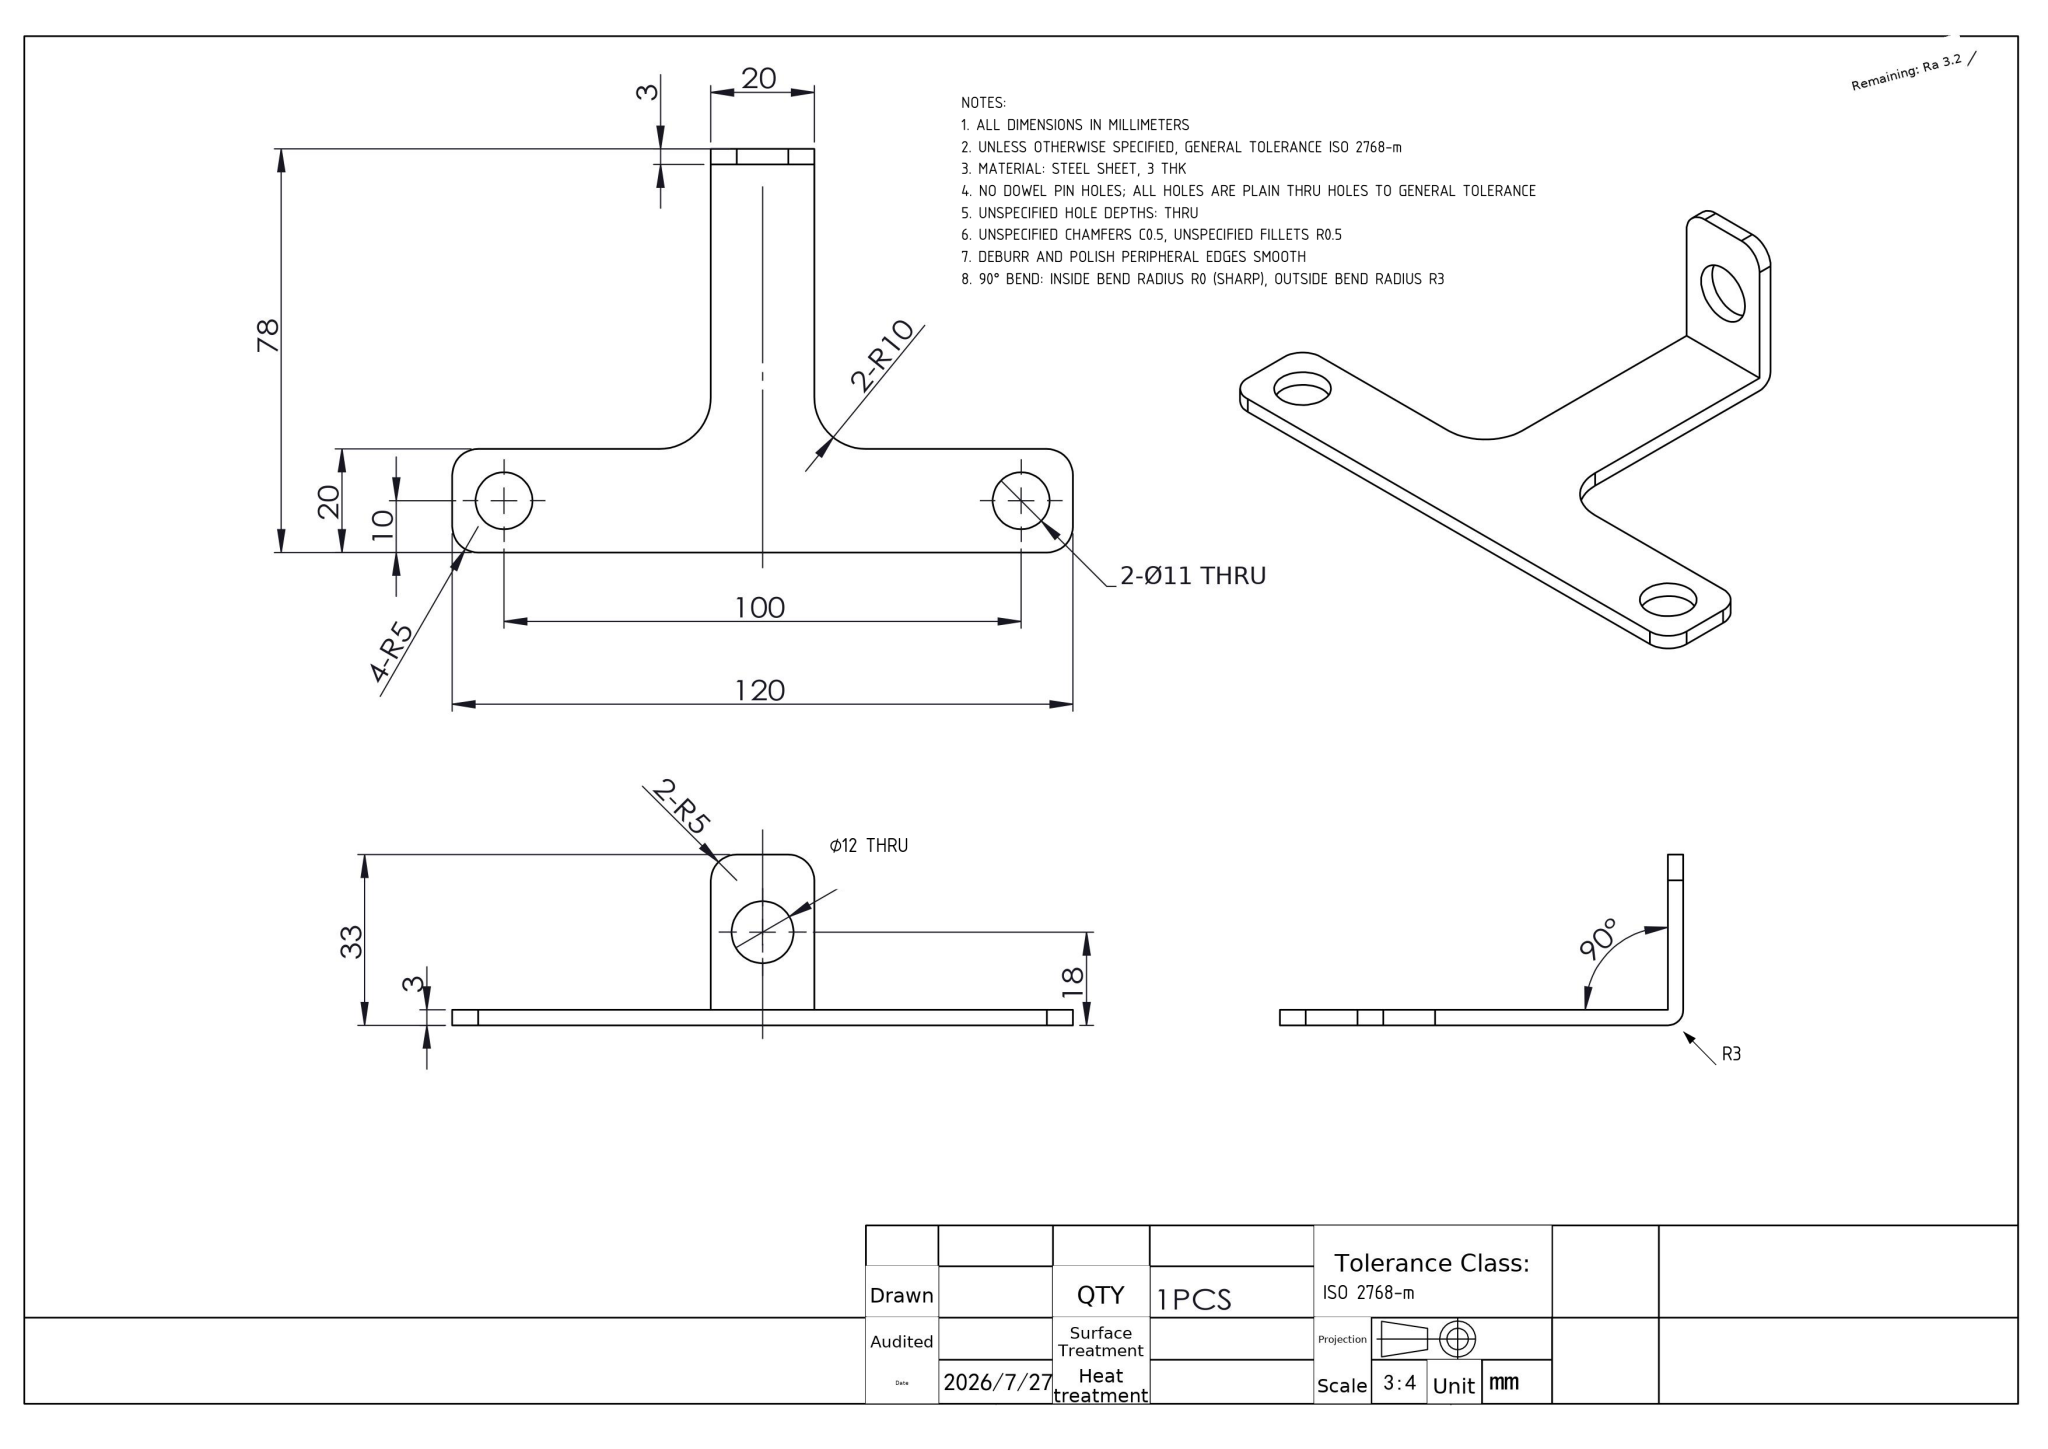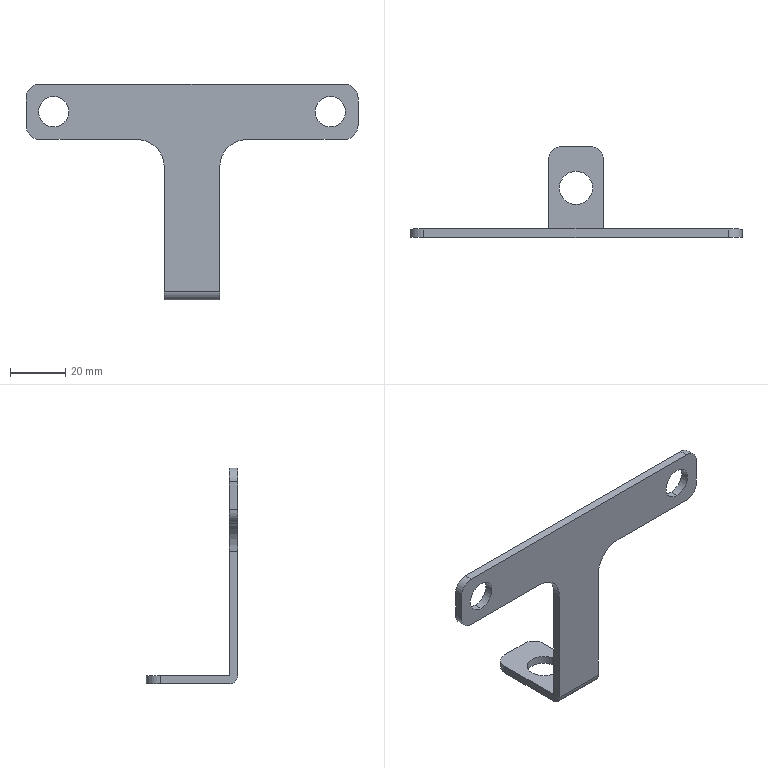Part | NX | mm | 1 solid | 27 faces | box 120 x 33 x 78 mm | volume 11564 mm3 | cylinder 15 | plane 12 | commonest cylinder face diameters 10 x6 11 x4 12 x2 20 x2 6 x1
STEP:
#1=COLOUR_RGB('',0.7922,0.8196,0.9333);
#2=FILL_AREA_STYLE_COLOUR('',#1);
#3=FILL_AREA_STYLE('',(#2));
#4=SURFACE_STYLE_FILL_AREA(#3);
#5=SURFACE_SIDE_STYLE('',(#4));
#6=SURFACE_STYLE_USAGE(.BOTH.,#5);
#7=PRESENTATION_STYLE_ASSIGNMENT((#6));
#8=CARTESIAN_POINT('',(-6.,15.,-75.));
#9=VERTEX_POINT('',#8);
#10=CARTESIAN_POINT('',(6.,15.,-75.));
#11=VERTEX_POINT('',#10);
#12=CARTESIAN_POINT('',(0.,15.,-75.));
#13=DIRECTION('',(0.,0.,1.));
#14=DIRECTION('',(1.,0.,0.));
#15=AXIS2_PLACEMENT_3D('',#12,#13,#14);
#16=CIRCLE('',#15,6.);
#17=EDGE_CURVE('',#9,#11,#16,.T.);
#18=ORIENTED_EDGE('',*,*,#17,.T.);
#19=CARTESIAN_POINT('',(6.,15.,-78.));
#20=VERTEX_POINT('',#19);
#21=CARTESIAN_POINT('',(6.,15.,0.));
#22=DIRECTION('',(0.,0.,-1.));
#23=VECTOR('',#22,1000.);
#24=LINE('',#21,#23);
#25=EDGE_CURVE('',#11,#20,#24,.T.);
#26=ORIENTED_EDGE('',*,*,#25,.T.);
#27=CARTESIAN_POINT('',(-6.,15.,-78.));
#28=VERTEX_POINT('',#27);
#29=CARTESIAN_POINT('',(0.,15.,-78.));
#30=DIRECTION('',(0.,0.,-1.));
#31=DIRECTION('',(-1.,0.,0.));
#32=AXIS2_PLACEMENT_3D('',#29,#30,#31);
#33=CIRCLE('',#32,6.);
#34=EDGE_CURVE('',#20,#28,#33,.T.);
#35=ORIENTED_EDGE('',*,*,#34,.T.);
#36=CARTESIAN_POINT('',(-6.,15.,0.));
#37=DIRECTION('',(0.,0.,-1.));
#38=VECTOR('',#37,1000.);
#39=LINE('',#36,#38);
#40=EDGE_CURVE('',#9,#28,#39,.T.);
#41=ORIENTED_EDGE('',*,*,#40,.F.);
#42=EDGE_LOOP('',(#18,#26,#35,#41));
#43=FACE_OUTER_BOUND('',#42,.T.);
#44=CARTESIAN_POINT('',(0.,15.,0.));
#45=DIRECTION('',(0.,0.,-1.));
#46=DIRECTION('',(-1.,0.,0.));
#47=AXIS2_PLACEMENT_3D('',#44,#45,#46);
#48=CYLINDRICAL_SURFACE('',#47,6.);
#49=ADVANCED_FACE('',(#43),#48,.F.);
#50=CARTESIAN_POINT('',(50.,-3.,-15.5));
#51=VERTEX_POINT('',#50);
#52=CARTESIAN_POINT('',(50.,-3.,-4.5));
#53=VERTEX_POINT('',#52);
#54=CARTESIAN_POINT('',(50.,-3.,-10.));
#55=DIRECTION('',(0.,1.,0.));
#56=DIRECTION('',(0.,0.,1.));
#57=AXIS2_PLACEMENT_3D('',#54,#55,#56);
#58=CIRCLE('',#57,5.5);
#59=EDGE_CURVE('',#51,#53,#58,.T.);
#60=ORIENTED_EDGE('',*,*,#59,.F.);
#61=CARTESIAN_POINT('',(50.,0.,-15.5));
#62=VERTEX_POINT('',#61);
#63=CARTESIAN_POINT('',(50.,-3.,-15.5));
#64=DIRECTION('',(0.,1.,0.));
#65=VECTOR('',#64,1000.);
#66=LINE('',#63,#65);
#67=EDGE_CURVE('',#51,#62,#66,.T.);
#68=ORIENTED_EDGE('',*,*,#67,.T.);
#69=CARTESIAN_POINT('',(50.,0.,-4.5));
#70=VERTEX_POINT('',#69);
#71=CARTESIAN_POINT('',(50.,0.,-10.));
#72=DIRECTION('',(0.,1.,0.));
#73=DIRECTION('',(0.,0.,1.));
#74=AXIS2_PLACEMENT_3D('',#71,#72,#73);
#75=CIRCLE('',#74,5.5);
#76=EDGE_CURVE('',#62,#70,#75,.T.);
#77=ORIENTED_EDGE('',*,*,#76,.T.);
#78=CARTESIAN_POINT('',(50.,-3.,-4.5));
#79=DIRECTION('',(0.,1.,0.));
#80=VECTOR('',#79,1000.);
#81=LINE('',#78,#80);
#82=EDGE_CURVE('',#53,#70,#81,.T.);
#83=ORIENTED_EDGE('',*,*,#82,.F.);
#84=EDGE_LOOP('',(#60,#68,#77,#83));
#85=FACE_OUTER_BOUND('',#84,.T.);
#86=CARTESIAN_POINT('',(50.,-3.,-10.));
#87=DIRECTION('',(0.,1.,0.));
#88=DIRECTION('',(0.,0.,1.));
#89=AXIS2_PLACEMENT_3D('',#86,#87,#88);
#90=CYLINDRICAL_SURFACE('',#89,5.5);
#91=ADVANCED_FACE('',(#85),#90,.F.);
#92=CARTESIAN_POINT('',(-50.,-3.,-15.5));
#93=VERTEX_POINT('',#92);
#94=CARTESIAN_POINT('',(-50.,-3.,-4.5));
#95=VERTEX_POINT('',#94);
#96=CARTESIAN_POINT('',(-50.,-3.,-10.));
#97=DIRECTION('',(0.,1.,0.));
#98=DIRECTION('',(0.,0.,-1.));
#99=AXIS2_PLACEMENT_3D('',#96,#97,#98);
#100=CIRCLE('',#99,5.5);
#101=EDGE_CURVE('',#93,#95,#100,.T.);
#102=ORIENTED_EDGE('',*,*,#101,.F.);
#103=CARTESIAN_POINT('',(-50.,0.,-15.5));
#104=VERTEX_POINT('',#103);
#105=CARTESIAN_POINT('',(-50.,-3.,-15.5));
#106=DIRECTION('',(0.,1.,0.));
#107=VECTOR('',#106,1000.);
#108=LINE('',#105,#107);
#109=EDGE_CURVE('',#93,#104,#108,.T.);
#110=ORIENTED_EDGE('',*,*,#109,.T.);
#111=CARTESIAN_POINT('',(-50.,0.,-4.5));
#112=VERTEX_POINT('',#111);
#113=CARTESIAN_POINT('',(-50.,0.,-10.));
#114=DIRECTION('',(0.,1.,0.));
#115=DIRECTION('',(0.,0.,-1.));
#116=AXIS2_PLACEMENT_3D('',#113,#114,#115);
#117=CIRCLE('',#116,5.5);
#118=EDGE_CURVE('',#104,#112,#117,.T.);
#119=ORIENTED_EDGE('',*,*,#118,.T.);
#120=CARTESIAN_POINT('',(-50.,-3.,-4.5));
#121=DIRECTION('',(0.,1.,0.));
#122=VECTOR('',#121,1000.);
#123=LINE('',#120,#122);
#124=EDGE_CURVE('',#95,#112,#123,.T.);
#125=ORIENTED_EDGE('',*,*,#124,.F.);
#126=EDGE_LOOP('',(#102,#110,#119,#125));
#127=FACE_OUTER_BOUND('',#126,.T.);
#128=CARTESIAN_POINT('',(-50.,-3.,-10.));
#129=DIRECTION('',(0.,1.,0.));
#130=DIRECTION('',(0.,0.,1.));
#131=AXIS2_PLACEMENT_3D('',#128,#129,#130);
#132=CYLINDRICAL_SURFACE('',#131,5.5);
#133=ADVANCED_FACE('',(#127),#132,.F.);
#134=CARTESIAN_POINT('',(60.,0.,-5.));
#135=VERTEX_POINT('',#134);
#136=CARTESIAN_POINT('',(60.,0.,-15.));
#137=VERTEX_POINT('',#136);
#138=CARTESIAN_POINT('',(60.,0.,0.));
#139=DIRECTION('',(0.,0.,-1.));
#140=VECTOR('',#139,1000.);
#141=LINE('',#138,#140);
#142=EDGE_CURVE('',#135,#137,#141,.T.);
#143=ORIENTED_EDGE('',*,*,#142,.F.);
#144=CARTESIAN_POINT('',(60.,-3.,-5.));
#145=VERTEX_POINT('',#144);
#146=CARTESIAN_POINT('',(60.,0.,-5.));
#147=DIRECTION('',(0.,-1.,0.));
#148=VECTOR('',#147,1000.);
#149=LINE('',#146,#148);
#150=EDGE_CURVE('',#135,#145,#149,.T.);
#151=ORIENTED_EDGE('',*,*,#150,.T.);
#152=CARTESIAN_POINT('',(60.,-3.,-15.));
#153=VERTEX_POINT('',#152);
#154=CARTESIAN_POINT('',(60.,-3.,0.));
#155=DIRECTION('',(0.,0.,-1.));
#156=VECTOR('',#155,1000.);
#157=LINE('',#154,#156);
#158=EDGE_CURVE('',#145,#153,#157,.T.);
#159=ORIENTED_EDGE('',*,*,#158,.T.);
#160=CARTESIAN_POINT('',(60.,0.,-15.));
#161=DIRECTION('',(0.,1.,0.));
#162=VECTOR('',#161,1000.);
#163=LINE('',#160,#162);
#164=EDGE_CURVE('',#153,#137,#163,.T.);
#165=ORIENTED_EDGE('',*,*,#164,.T.);
#166=EDGE_LOOP('',(#143,#151,#159,#165));
#167=FACE_OUTER_BOUND('',#166,.T.);
#168=CARTESIAN_POINT('',(60.,0.,-75.));
#169=DIRECTION('',(1.,0.,0.));
#170=DIRECTION('',(0.,0.,-1.));
#171=AXIS2_PLACEMENT_3D('',#168,#169,#170);
#172=PLANE('',#171);
#173=ADVANCED_FACE('',(#167),#172,.T.);
#174=CARTESIAN_POINT('',(0.,15.,-78.));
#175=DIRECTION('',(0.,0.,-1.));
#176=DIRECTION('',(-1.,0.,0.));
#177=AXIS2_PLACEMENT_3D('',#174,#175,#176);
#178=CIRCLE('',#177,6.);
#179=EDGE_CURVE('',#28,#20,#178,.T.);
#180=ORIENTED_EDGE('',*,*,#179,.F.);
#181=ORIENTED_EDGE('',*,*,#34,.F.);
#182=EDGE_LOOP('',(#180,#181));
#183=FACE_BOUND('',#182,.T.);
#184=CARTESIAN_POINT('',(-10.,0.,-78.));
#185=VERTEX_POINT('',#184);
#186=CARTESIAN_POINT('',(-10.,25.,-78.));
#187=VERTEX_POINT('',#186);
#188=CARTESIAN_POINT('',(-10.,-3.,-78.));
#189=DIRECTION('',(0.,1.,0.));
#190=VECTOR('',#189,1000.);
#191=LINE('',#188,#190);
#192=EDGE_CURVE('',#185,#187,#191,.T.);
#193=ORIENTED_EDGE('',*,*,#192,.T.);
#194=CARTESIAN_POINT('',(-5.,30.,-78.));
#195=VERTEX_POINT('',#194);
#196=CARTESIAN_POINT('',(-5.,25.,-78.));
#197=DIRECTION('',(0.,0.,-1.));
#198=DIRECTION('',(1.,0.,0.));
#199=AXIS2_PLACEMENT_3D('',#196,#197,#198);
#200=CIRCLE('',#199,5.);
#201=EDGE_CURVE('',#187,#195,#200,.T.);
#202=ORIENTED_EDGE('',*,*,#201,.T.);
#203=CARTESIAN_POINT('',(5.,30.,-78.));
#204=VERTEX_POINT('',#203);
#205=CARTESIAN_POINT('',(60.,30.,-78.));
#206=DIRECTION('',(-1.,0.,0.));
#207=VECTOR('',#206,1000.);
#208=LINE('',#205,#207);
#209=EDGE_CURVE('',#204,#195,#208,.T.);
#210=ORIENTED_EDGE('',*,*,#209,.F.);
#211=CARTESIAN_POINT('',(10.,25.,-78.));
#212=VERTEX_POINT('',#211);
#213=CARTESIAN_POINT('',(5.,25.,-78.));
#214=DIRECTION('',(0.,0.,-1.));
#215=DIRECTION('',(1.,-0.,0.));
#216=AXIS2_PLACEMENT_3D('',#213,#214,#215);
#217=CIRCLE('',#216,5.);
#218=EDGE_CURVE('',#204,#212,#217,.T.);
#219=ORIENTED_EDGE('',*,*,#218,.T.);
#220=CARTESIAN_POINT('',(10.,0.,-78.));
#221=VERTEX_POINT('',#220);
#222=CARTESIAN_POINT('',(10.,-3.,-78.));
#223=DIRECTION('',(0.,1.,0.));
#224=VECTOR('',#223,1000.);
#225=LINE('',#222,#224);
#226=EDGE_CURVE('',#221,#212,#225,.T.);
#227=ORIENTED_EDGE('',*,*,#226,.F.);
#228=CARTESIAN_POINT('',(60.,0.,-78.));
#229=DIRECTION('',(-1.,0.,0.));
#230=VECTOR('',#229,1000.);
#231=LINE('',#228,#230);
#232=EDGE_CURVE('',#221,#185,#231,.T.);
#233=ORIENTED_EDGE('',*,*,#232,.T.);
#234=EDGE_LOOP('',(#193,#202,#210,#219,#227,#233));
#235=FACE_OUTER_BOUND('',#234,.T.);
#236=CARTESIAN_POINT('',(60.,0.,-78.));
#237=DIRECTION('',(0.,0.,1.));
#238=DIRECTION('',(1.,0.,0.));
#239=AXIS2_PLACEMENT_3D('',#236,#237,#238);
#240=PLANE('',#239);
#241=ADVANCED_FACE('',(#183,#235),#240,.F.);
#242=ORIENTED_EDGE('',*,*,#209,.T.);
#243=CARTESIAN_POINT('',(-5.,30.,-75.));
#244=VERTEX_POINT('',#243);
#245=CARTESIAN_POINT('',(-5.,30.,-75.));
#246=DIRECTION('',(-0.,0.,1.));
#247=VECTOR('',#246,1000.);
#248=LINE('',#245,#247);
#249=EDGE_CURVE('',#195,#244,#248,.T.);
#250=ORIENTED_EDGE('',*,*,#249,.T.);
#251=CARTESIAN_POINT('',(5.,30.,-75.));
#252=VERTEX_POINT('',#251);
#253=CARTESIAN_POINT('',(60.,30.,-75.));
#254=DIRECTION('',(-1.,0.,0.));
#255=VECTOR('',#254,1000.);
#256=LINE('',#253,#255);
#257=EDGE_CURVE('',#252,#244,#256,.T.);
#258=ORIENTED_EDGE('',*,*,#257,.F.);
#259=CARTESIAN_POINT('',(5.,30.,-78.));
#260=DIRECTION('',(-0.,0.,-1.));
#261=VECTOR('',#260,1000.);
#262=LINE('',#259,#261);
#263=EDGE_CURVE('',#252,#204,#262,.T.);
#264=ORIENTED_EDGE('',*,*,#263,.T.);
#265=EDGE_LOOP('',(#242,#250,#258,#264));
#266=FACE_OUTER_BOUND('',#265,.T.);
#267=CARTESIAN_POINT('',(60.,30.,-75.));
#268=DIRECTION('',(0.,1.,0.));
#269=DIRECTION('',(0.,0.,1.));
#270=AXIS2_PLACEMENT_3D('',#267,#268,#269);
#271=PLANE('',#270);
#272=ADVANCED_FACE('',(#266),#271,.T.);
#273=ORIENTED_EDGE('',*,*,#17,.F.);
#274=CARTESIAN_POINT('',(0.,15.,-75.));
#275=DIRECTION('',(0.,0.,1.));
#276=DIRECTION('',(1.,0.,0.));
#277=AXIS2_PLACEMENT_3D('',#274,#275,#276);
#278=CIRCLE('',#277,6.);
#279=EDGE_CURVE('',#11,#9,#278,.T.);
#280=ORIENTED_EDGE('',*,*,#279,.F.);
#281=EDGE_LOOP('',(#273,#280));
#282=FACE_BOUND('',#281,.T.);
#283=ORIENTED_EDGE('',*,*,#257,.T.);
#284=CARTESIAN_POINT('',(-10.,25.,-75.));
#285=VERTEX_POINT('',#284);
#286=CARTESIAN_POINT('',(-5.,25.,-75.));
#287=DIRECTION('',(0.,0.,1.));
#288=DIRECTION('',(1.,0.,0.));
#289=AXIS2_PLACEMENT_3D('',#286,#287,#288);
#290=CIRCLE('',#289,5.);
#291=EDGE_CURVE('',#244,#285,#290,.T.);
#292=ORIENTED_EDGE('',*,*,#291,.T.);
#293=CARTESIAN_POINT('',(-10.,0.,-75.));
#294=VERTEX_POINT('',#293);
#295=CARTESIAN_POINT('',(-10.,0.,-75.));
#296=DIRECTION('',(0.,1.,0.));
#297=VECTOR('',#296,1000.);
#298=LINE('',#295,#297);
#299=EDGE_CURVE('',#294,#285,#298,.T.);
#300=ORIENTED_EDGE('',*,*,#299,.F.);
#301=CARTESIAN_POINT('',(10.,0.,-75.));
#302=VERTEX_POINT('',#301);
#303=CARTESIAN_POINT('',(60.,0.,-75.));
#304=DIRECTION('',(-1.,0.,0.));
#305=VECTOR('',#304,1000.);
#306=LINE('',#303,#305);
#307=EDGE_CURVE('',#302,#294,#306,.T.);
#308=ORIENTED_EDGE('',*,*,#307,.F.);
#309=CARTESIAN_POINT('',(10.,25.,-75.));
#310=VERTEX_POINT('',#309);
#311=CARTESIAN_POINT('',(10.,0.,-75.));
#312=DIRECTION('',(0.,-1.,0.));
#313=VECTOR('',#312,1000.);
#314=LINE('',#311,#313);
#315=EDGE_CURVE('',#310,#302,#314,.T.);
#316=ORIENTED_EDGE('',*,*,#315,.F.);
#317=CARTESIAN_POINT('',(5.,25.,-75.));
#318=DIRECTION('',(0.,0.,1.));
#319=DIRECTION('',(1.,0.,0.));
#320=AXIS2_PLACEMENT_3D('',#317,#318,#319);
#321=CIRCLE('',#320,5.);
#322=EDGE_CURVE('',#310,#252,#321,.T.);
#323=ORIENTED_EDGE('',*,*,#322,.T.);
#324=EDGE_LOOP('',(#283,#292,#300,#308,#316,#323));
#325=FACE_OUTER_BOUND('',#324,.T.);
#326=CARTESIAN_POINT('',(60.,0.,-75.));
#327=DIRECTION('',(0.,0.,1.));
#328=DIRECTION('',(1.,0.,0.));
#329=AXIS2_PLACEMENT_3D('',#326,#327,#328);
#330=PLANE('',#329);
#331=ADVANCED_FACE('',(#282,#325),#330,.T.);
#332=CARTESIAN_POINT('',(50.,0.,-10.));
#333=DIRECTION('',(0.,1.,0.));
#334=DIRECTION('',(0.,0.,1.));
#335=AXIS2_PLACEMENT_3D('',#332,#333,#334);
#336=CIRCLE('',#335,5.5);
#337=EDGE_CURVE('',#70,#62,#336,.T.);
#338=ORIENTED_EDGE('',*,*,#337,.F.);
#339=ORIENTED_EDGE('',*,*,#76,.F.);
#340=EDGE_LOOP('',(#338,#339));
#341=FACE_BOUND('',#340,.T.);
#342=CARTESIAN_POINT('',(-50.,0.,-10.));
#343=DIRECTION('',(0.,1.,0.));
#344=DIRECTION('',(0.,0.,-1.));
#345=AXIS2_PLACEMENT_3D('',#342,#343,#344);
#346=CIRCLE('',#345,5.5);
#347=EDGE_CURVE('',#112,#104,#346,.T.);
#348=ORIENTED_EDGE('',*,*,#347,.F.);
#349=ORIENTED_EDGE('',*,*,#118,.F.);
#350=EDGE_LOOP('',(#348,#349));
#351=FACE_BOUND('',#350,.T.);
#352=CARTESIAN_POINT('',(-60.,0.,-5.));
#353=VERTEX_POINT('',#352);
#354=CARTESIAN_POINT('',(-60.,0.,-15.));
#355=VERTEX_POINT('',#354);
#356=CARTESIAN_POINT('',(-60.,0.,0.));
#357=DIRECTION('',(0.,0.,-1.));
#358=VECTOR('',#357,1000.);
#359=LINE('',#356,#358);
#360=EDGE_CURVE('',#353,#355,#359,.T.);
#361=ORIENTED_EDGE('',*,*,#360,.F.);
#362=CARTESIAN_POINT('',(-55.,0.,0.));
#363=VERTEX_POINT('',#362);
#364=CARTESIAN_POINT('',(-55.,0.,-5.));
#365=DIRECTION('',(0.,1.,0.));
#366=DIRECTION('',(0.,0.,1.));
#367=AXIS2_PLACEMENT_3D('',#364,#365,#366);
#368=CIRCLE('',#367,5.);
#369=EDGE_CURVE('',#353,#363,#368,.T.);
#370=ORIENTED_EDGE('',*,*,#369,.T.);
#371=CARTESIAN_POINT('',(55.,0.,0.));
#372=VERTEX_POINT('',#371);
#373=CARTESIAN_POINT('',(60.,0.,0.));
#374=DIRECTION('',(-1.,0.,0.));
#375=VECTOR('',#374,1000.);
#376=LINE('',#373,#375);
#377=EDGE_CURVE('',#372,#363,#376,.T.);
#378=ORIENTED_EDGE('',*,*,#377,.F.);
#379=CARTESIAN_POINT('',(55.,0.,-5.));
#380=DIRECTION('',(0.,1.,0.));
#381=DIRECTION('',(0.,0.,1.));
#382=AXIS2_PLACEMENT_3D('',#379,#380,#381);
#383=CIRCLE('',#382,5.);
#384=EDGE_CURVE('',#372,#135,#383,.T.);
#385=ORIENTED_EDGE('',*,*,#384,.T.);
#386=ORIENTED_EDGE('',*,*,#142,.T.);
#387=CARTESIAN_POINT('',(55.,0.,-20.));
#388=VERTEX_POINT('',#387);
#389=CARTESIAN_POINT('',(55.,0.,-15.));
#390=DIRECTION('',(0.,1.,0.));
#391=DIRECTION('',(0.,0.,1.));
#392=AXIS2_PLACEMENT_3D('',#389,#390,#391);
#393=CIRCLE('',#392,5.);
#394=EDGE_CURVE('',#137,#388,#393,.T.);
#395=ORIENTED_EDGE('',*,*,#394,.T.);
#396=CARTESIAN_POINT('',(20.,0.,-20.));
#397=VERTEX_POINT('',#396);
#398=CARTESIAN_POINT('',(60.,0.,-20.));
#399=DIRECTION('',(1.,0.,-0.));
#400=VECTOR('',#399,1000.);
#401=LINE('',#398,#400);
#402=EDGE_CURVE('',#397,#388,#401,.T.);
#403=ORIENTED_EDGE('',*,*,#402,.F.);
#404=CARTESIAN_POINT('',(10.,0.,-30.));
#405=VERTEX_POINT('',#404);
#406=CARTESIAN_POINT('',(20.,0.,-30.));
#407=DIRECTION('',(0.,-1.,0.));
#408=DIRECTION('',(0.,0.,1.));
#409=AXIS2_PLACEMENT_3D('',#406,#407,#408);
#410=CIRCLE('',#409,10.);
#411=EDGE_CURVE('',#397,#405,#410,.T.);
#412=ORIENTED_EDGE('',*,*,#411,.T.);
#413=CARTESIAN_POINT('',(10.,0.,0.));
#414=DIRECTION('',(0.,0.,1.));
#415=VECTOR('',#414,1000.);
#416=LINE('',#413,#415);
#417=EDGE_CURVE('',#302,#405,#416,.T.);
#418=ORIENTED_EDGE('',*,*,#417,.F.);
#419=ORIENTED_EDGE('',*,*,#307,.T.);
#420=CARTESIAN_POINT('',(-10.,0.,-30.));
#421=VERTEX_POINT('',#420);
#422=CARTESIAN_POINT('',(-10.,0.,-0.));
#423=DIRECTION('',(0.,0.,-1.));
#424=VECTOR('',#423,1000.);
#425=LINE('',#422,#424);
#426=EDGE_CURVE('',#421,#294,#425,.T.);
#427=ORIENTED_EDGE('',*,*,#426,.F.);
#428=CARTESIAN_POINT('',(-20.,0.,-20.));
#429=VERTEX_POINT('',#428);
#430=CARTESIAN_POINT('',(-20.,0.,-30.));
#431=DIRECTION('',(0.,-1.,0.));
#432=DIRECTION('',(-0.,0.,1.));
#433=AXIS2_PLACEMENT_3D('',#430,#431,#432);
#434=CIRCLE('',#433,10.);
#435=EDGE_CURVE('',#421,#429,#434,.T.);
#436=ORIENTED_EDGE('',*,*,#435,.T.);
#437=CARTESIAN_POINT('',(-55.,0.,-20.));
#438=VERTEX_POINT('',#437);
#439=CARTESIAN_POINT('',(60.,0.,-20.));
#440=DIRECTION('',(1.,0.,0.));
#441=VECTOR('',#440,1000.);
#442=LINE('',#439,#441);
#443=EDGE_CURVE('',#438,#429,#442,.T.);
#444=ORIENTED_EDGE('',*,*,#443,.F.);
#445=CARTESIAN_POINT('',(-55.,0.,-15.));
#446=DIRECTION('',(0.,1.,0.));
#447=DIRECTION('',(0.,0.,1.));
#448=AXIS2_PLACEMENT_3D('',#445,#446,#447);
#449=CIRCLE('',#448,5.);
#450=EDGE_CURVE('',#438,#355,#449,.T.);
#451=ORIENTED_EDGE('',*,*,#450,.T.);
#452=EDGE_LOOP('',(#361,#370,#378,#385,#386,#395,#403,#412,#418,#419,#427,#436,#444,#451));
#453=FACE_OUTER_BOUND('',#452,.T.);
#454=CARTESIAN_POINT('',(60.,0.,0.));
#455=DIRECTION('',(0.,1.,0.));
#456=DIRECTION('',(0.,0.,1.));
#457=AXIS2_PLACEMENT_3D('',#454,#455,#456);
#458=PLANE('',#457);
#459=ADVANCED_FACE('',(#341,#351,#453),#458,.T.);
#460=ORIENTED_EDGE('',*,*,#377,.T.);
#461=CARTESIAN_POINT('',(-55.,-3.,0.));
#462=VERTEX_POINT('',#461);
#463=CARTESIAN_POINT('',(-55.,-3.,0.));
#464=DIRECTION('',(0.,-1.,0.));
#465=VECTOR('',#464,1000.);
#466=LINE('',#463,#465);
#467=EDGE_CURVE('',#363,#462,#466,.T.);
#468=ORIENTED_EDGE('',*,*,#467,.T.);
#469=CARTESIAN_POINT('',(55.,-3.,0.));
#470=VERTEX_POINT('',#469);
#471=CARTESIAN_POINT('',(60.,-3.,0.));
#472=DIRECTION('',(-1.,0.,0.));
#473=VECTOR('',#472,1000.);
#474=LINE('',#471,#473);
#475=EDGE_CURVE('',#470,#462,#474,.T.);
#476=ORIENTED_EDGE('',*,*,#475,.F.);
#477=CARTESIAN_POINT('',(55.,-3.,0.));
#478=DIRECTION('',(0.,1.,0.));
#479=VECTOR('',#478,1000.);
#480=LINE('',#477,#479);
#481=EDGE_CURVE('',#470,#372,#480,.T.);
#482=ORIENTED_EDGE('',*,*,#481,.T.);
#483=EDGE_LOOP('',(#460,#468,#476,#482));
#484=FACE_OUTER_BOUND('',#483,.T.);
#485=CARTESIAN_POINT('',(60.,-3.,0.));
#486=DIRECTION('',(0.,0.,1.));
#487=DIRECTION('',(1.,0.,0.));
#488=AXIS2_PLACEMENT_3D('',#485,#486,#487);
#489=PLANE('',#488);
#490=ADVANCED_FACE('',(#484),#489,.T.);
#491=CARTESIAN_POINT('',(50.,-3.,-10.));
#492=DIRECTION('',(0.,1.,0.));
#493=DIRECTION('',(0.,0.,1.));
#494=AXIS2_PLACEMENT_3D('',#491,#492,#493);
#495=CIRCLE('',#494,5.5);
#496=EDGE_CURVE('',#53,#51,#495,.T.);
#497=ORIENTED_EDGE('',*,*,#496,.T.);
#498=ORIENTED_EDGE('',*,*,#59,.T.);
#499=EDGE_LOOP('',(#497,#498));
#500=FACE_BOUND('',#499,.T.);
#501=CARTESIAN_POINT('',(-50.,-3.,-10.));
#502=DIRECTION('',(0.,1.,0.));
#503=DIRECTION('',(0.,0.,-1.));
#504=AXIS2_PLACEMENT_3D('',#501,#502,#503);
#505=CIRCLE('',#504,5.5);
#506=EDGE_CURVE('',#95,#93,#505,.T.);
#507=ORIENTED_EDGE('',*,*,#506,.T.);
#508=ORIENTED_EDGE('',*,*,#101,.T.);
#509=EDGE_LOOP('',(#507,#508));
#510=FACE_BOUND('',#509,.T.);
#511=ORIENTED_EDGE('',*,*,#475,.T.);
#512=CARTESIAN_POINT('',(-60.,-3.,-5.));
#513=VERTEX_POINT('',#512);
#514=CARTESIAN_POINT('',(-55.,-3.,-5.));
#515=DIRECTION('',(0.,-1.,0.));
#516=DIRECTION('',(0.,0.,1.));
#517=AXIS2_PLACEMENT_3D('',#514,#515,#516);
#518=CIRCLE('',#517,5.);
#519=EDGE_CURVE('',#462,#513,#518,.T.);
#520=ORIENTED_EDGE('',*,*,#519,.T.);
#521=CARTESIAN_POINT('',(-60.,-3.,-15.));
#522=VERTEX_POINT('',#521);
#523=CARTESIAN_POINT('',(-60.,-3.,0.));
#524=DIRECTION('',(0.,0.,-1.));
#525=VECTOR('',#524,1000.);
#526=LINE('',#523,#525);
#527=EDGE_CURVE('',#513,#522,#526,.T.);
#528=ORIENTED_EDGE('',*,*,#527,.T.);
#529=CARTESIAN_POINT('',(-55.,-3.,-20.));
#530=VERTEX_POINT('',#529);
#531=CARTESIAN_POINT('',(-55.,-3.,-15.));
#532=DIRECTION('',(0.,-1.,0.));
#533=DIRECTION('',(0.,0.,1.));
#534=AXIS2_PLACEMENT_3D('',#531,#532,#533);
#535=CIRCLE('',#534,5.);
#536=EDGE_CURVE('',#522,#530,#535,.T.);
#537=ORIENTED_EDGE('',*,*,#536,.T.);
#538=CARTESIAN_POINT('',(-20.,-3.,-20.));
#539=VERTEX_POINT('',#538);
#540=CARTESIAN_POINT('',(-60.,-3.,-20.));
#541=DIRECTION('',(1.,0.,0.));
#542=VECTOR('',#541,1000.);
#543=LINE('',#540,#542);
#544=EDGE_CURVE('',#530,#539,#543,.T.);
#545=ORIENTED_EDGE('',*,*,#544,.T.);
#546=CARTESIAN_POINT('',(-10.,-3.,-30.));
#547=VERTEX_POINT('',#546);
#548=CARTESIAN_POINT('',(-20.,-3.,-30.));
#549=DIRECTION('',(0.,1.,0.));
#550=DIRECTION('',(0.,0.,1.));
#551=AXIS2_PLACEMENT_3D('',#548,#549,#550);
#552=CIRCLE('',#551,10.);
#553=EDGE_CURVE('',#539,#547,#552,.T.);
#554=ORIENTED_EDGE('',*,*,#553,.T.);
#555=CARTESIAN_POINT('',(-10.,-3.,-75.));
#556=VERTEX_POINT('',#555);
#557=CARTESIAN_POINT('',(-10.,-3.,-78.));
#558=DIRECTION('',(0.,0.,-1.));
#559=VECTOR('',#558,1000.);
#560=LINE('',#557,#559);
#561=EDGE_CURVE('',#547,#556,#560,.T.);
#562=ORIENTED_EDGE('',*,*,#561,.T.);
#563=CARTESIAN_POINT('',(10.,-3.,-75.));
#564=VERTEX_POINT('',#563);
#565=CARTESIAN_POINT('',(60.,-3.,-75.));
#566=DIRECTION('',(1.,0.,0.));
#567=VECTOR('',#566,1000.);
#568=LINE('',#565,#567);
#569=EDGE_CURVE('',#556,#564,#568,.T.);
#570=ORIENTED_EDGE('',*,*,#569,.T.);
#571=CARTESIAN_POINT('',(10.,-3.,-30.));
#572=VERTEX_POINT('',#571);
#573=CARTESIAN_POINT('',(10.,-3.,-78.));
#574=DIRECTION('',(0.,0.,1.));
#575=VECTOR('',#574,1000.);
#576=LINE('',#573,#575);
#577=EDGE_CURVE('',#564,#572,#576,.T.);
#578=ORIENTED_EDGE('',*,*,#577,.T.);
#579=CARTESIAN_POINT('',(20.,-3.,-20.));
#580=VERTEX_POINT('',#579);
#581=CARTESIAN_POINT('',(20.,-3.,-30.));
#582=DIRECTION('',(0.,1.,0.));
#583=DIRECTION('',(0.,0.,1.));
#584=AXIS2_PLACEMENT_3D('',#581,#582,#583);
#585=CIRCLE('',#584,10.);
#586=EDGE_CURVE('',#572,#580,#585,.T.);
#587=ORIENTED_EDGE('',*,*,#586,.T.);
#588=CARTESIAN_POINT('',(55.,-3.,-20.));
#589=VERTEX_POINT('',#588);
#590=CARTESIAN_POINT('',(60.,-3.,-20.));
#591=DIRECTION('',(1.,0.,-0.));
#592=VECTOR('',#591,1000.);
#593=LINE('',#590,#592);
#594=EDGE_CURVE('',#580,#589,#593,.T.);
#595=ORIENTED_EDGE('',*,*,#594,.T.);
#596=CARTESIAN_POINT('',(55.,-3.,-15.));
#597=DIRECTION('',(0.,-1.,0.));
#598=DIRECTION('',(0.,0.,1.));
#599=AXIS2_PLACEMENT_3D('',#596,#597,#598);
#600=CIRCLE('',#599,5.);
#601=EDGE_CURVE('',#589,#153,#600,.T.);
#602=ORIENTED_EDGE('',*,*,#601,.T.);
#603=ORIENTED_EDGE('',*,*,#158,.F.);
#604=CARTESIAN_POINT('',(55.,-3.,-5.));
#605=DIRECTION('',(0.,-1.,0.));
#606=DIRECTION('',(0.,0.,1.));
#607=AXIS2_PLACEMENT_3D('',#604,#605,#606);
#608=CIRCLE('',#607,5.);
#609=EDGE_CURVE('',#145,#470,#608,.T.);
#610=ORIENTED_EDGE('',*,*,#609,.T.);
#611=EDGE_LOOP('',(#511,#520,#528,#537,#545,#554,#562,#570,#578,#587,#595,#602,#603,#610));
#612=FACE_OUTER_BOUND('',#611,.T.);
#613=CARTESIAN_POINT('',(60.,-3.,0.));
#614=DIRECTION('',(0.,1.,0.));
#615=DIRECTION('',(0.,0.,1.));
#616=AXIS2_PLACEMENT_3D('',#613,#614,#615);
#617=PLANE('',#616);
#618=ADVANCED_FACE('',(#500,#510,#612),#617,.F.);
#619=ORIENTED_EDGE('',*,*,#527,.F.);
#620=CARTESIAN_POINT('',(-60.,0.,-5.));
#621=DIRECTION('',(0.,1.,0.));
#622=VECTOR('',#621,1000.);
#623=LINE('',#620,#622);
#624=EDGE_CURVE('',#513,#353,#623,.T.);
#625=ORIENTED_EDGE('',*,*,#624,.T.);
#626=ORIENTED_EDGE('',*,*,#360,.T.);
#627=CARTESIAN_POINT('',(-60.,-3.,-15.));
#628=DIRECTION('',(0.,-1.,0.));
#629=VECTOR('',#628,1000.);
#630=LINE('',#627,#629);
#631=EDGE_CURVE('',#355,#522,#630,.T.);
#632=ORIENTED_EDGE('',*,*,#631,.T.);
#633=EDGE_LOOP('',(#619,#625,#626,#632));
#634=FACE_OUTER_BOUND('',#633,.T.);
#635=CARTESIAN_POINT('',(-60.,0.,0.));
#636=DIRECTION('',(-1.,0.,0.));
#637=DIRECTION('',(0.,0.,1.));
#638=AXIS2_PLACEMENT_3D('',#635,#636,#637);
#639=PLANE('',#638);
#640=ADVANCED_FACE('',(#634),#639,.T.);
#641=CARTESIAN_POINT('',(10.,0.,-75.));
#642=DIRECTION('',(1.,0.,-0.));
#643=DIRECTION('',(0.,0.,1.));
#644=AXIS2_PLACEMENT_3D('',#641,#642,#643);
#645=CIRCLE('',#644,3.);
#646=EDGE_CURVE('',#564,#221,#645,.T.);
#647=ORIENTED_EDGE('',*,*,#646,.F.);
#648=ORIENTED_EDGE('',*,*,#569,.F.);
#649=CARTESIAN_POINT('',(-10.,0.,-75.));
#650=DIRECTION('',(-1.,0.,-0.));
#651=DIRECTION('',(0.,0.,-1.));
#652=AXIS2_PLACEMENT_3D('',#649,#650,#651);
#653=CIRCLE('',#652,3.);
#654=EDGE_CURVE('',#185,#556,#653,.T.);
#655=ORIENTED_EDGE('',*,*,#654,.F.);
#656=ORIENTED_EDGE('',*,*,#232,.F.);
#657=EDGE_LOOP('',(#647,#648,#655,#656));
#658=FACE_OUTER_BOUND('',#657,.T.);
#659=CARTESIAN_POINT('',(60.,0.,-75.));
#660=DIRECTION('',(-1.,0.,0.));
#661=DIRECTION('',(0.,0.,1.));
#662=AXIS2_PLACEMENT_3D('',#659,#660,#661);
#663=CYLINDRICAL_SURFACE('',#662,3.);
#664=ADVANCED_FACE('',(#658),#663,.T.);
#665=ORIENTED_EDGE('',*,*,#299,.T.);
#666=CARTESIAN_POINT('',(-10.,25.,-78.));
#667=DIRECTION('',(0.,0.,-1.));
#668=VECTOR('',#667,1000.);
#669=LINE('',#666,#668);
#670=EDGE_CURVE('',#285,#187,#669,.T.);
#671=ORIENTED_EDGE('',*,*,#670,.T.);
#672=ORIENTED_EDGE('',*,*,#192,.F.);
#673=ORIENTED_EDGE('',*,*,#654,.T.);
#674=ORIENTED_EDGE('',*,*,#561,.F.);
#675=CARTESIAN_POINT('',(-10.,0.,-30.));
#676=DIRECTION('',(0.,1.,0.));
#677=VECTOR('',#676,1000.);
#678=LINE('',#675,#677);
#679=EDGE_CURVE('',#547,#421,#678,.T.);
#680=ORIENTED_EDGE('',*,*,#679,.T.);
#681=ORIENTED_EDGE('',*,*,#426,.T.);
#682=EDGE_LOOP('',(#665,#671,#672,#673,#674,#680,#681));
#683=FACE_OUTER_BOUND('',#682,.T.);
#684=CARTESIAN_POINT('',(-10.,-3.,-78.));
#685=DIRECTION('',(1.,0.,0.));
#686=DIRECTION('',(0.,0.,-1.));
#687=AXIS2_PLACEMENT_3D('',#684,#685,#686);
#688=PLANE('',#687);
#689=ADVANCED_FACE('',(#683),#688,.F.);
#690=ORIENTED_EDGE('',*,*,#544,.F.);
#691=CARTESIAN_POINT('',(-55.,0.,-20.));
#692=DIRECTION('',(0.,1.,0.));
#693=VECTOR('',#692,1000.);
#694=LINE('',#691,#693);
#695=EDGE_CURVE('',#530,#438,#694,.T.);
#696=ORIENTED_EDGE('',*,*,#695,.T.);
#697=ORIENTED_EDGE('',*,*,#443,.T.);
#698=CARTESIAN_POINT('',(-20.,-3.,-20.));
#699=DIRECTION('',(0.,-1.,0.));
#700=VECTOR('',#699,1000.);
#701=LINE('',#698,#700);
#702=EDGE_CURVE('',#429,#539,#701,.T.);
#703=ORIENTED_EDGE('',*,*,#702,.T.);
#704=EDGE_LOOP('',(#690,#696,#697,#703));
#705=FACE_OUTER_BOUND('',#704,.T.);
#706=CARTESIAN_POINT('',(-60.,-3.,-20.));
#707=DIRECTION('',(-0.,0.,1.));
#708=DIRECTION('',(1.,0.,0.));
#709=AXIS2_PLACEMENT_3D('',#706,#707,#708);
#710=PLANE('',#709);
#711=ADVANCED_FACE('',(#705),#710,.F.);
#712=ORIENTED_EDGE('',*,*,#402,.T.);
#713=CARTESIAN_POINT('',(55.,-3.,-20.));
#714=DIRECTION('',(0.,-1.,0.));
#715=VECTOR('',#714,1000.);
#716=LINE('',#713,#715);
#717=EDGE_CURVE('',#388,#589,#716,.T.);
#718=ORIENTED_EDGE('',*,*,#717,.T.);
#719=ORIENTED_EDGE('',*,*,#594,.F.);
#720=CARTESIAN_POINT('',(20.,0.,-20.));
#721=DIRECTION('',(0.,1.,0.));
#722=VECTOR('',#721,1000.);
#723=LINE('',#720,#722);
#724=EDGE_CURVE('',#580,#397,#723,.T.);
#725=ORIENTED_EDGE('',*,*,#724,.T.);
#726=EDGE_LOOP('',(#712,#718,#719,#725));
#727=FACE_OUTER_BOUND('',#726,.T.);
#728=CARTESIAN_POINT('',(60.,-3.,-20.));
#729=DIRECTION('',(0.,0.,1.));
#730=DIRECTION('',(1.,0.,-0.));
#731=AXIS2_PLACEMENT_3D('',#728,#729,#730);
#732=PLANE('',#731);
#733=ADVANCED_FACE('',(#727),#732,.F.);
#734=ORIENTED_EDGE('',*,*,#226,.T.);
#735=CARTESIAN_POINT('',(10.,25.,-75.));
#736=DIRECTION('',(0.,0.,1.));
#737=VECTOR('',#736,1000.);
#738=LINE('',#735,#737);
#739=EDGE_CURVE('',#212,#310,#738,.T.);
#740=ORIENTED_EDGE('',*,*,#739,.T.);
#741=ORIENTED_EDGE('',*,*,#315,.T.);
#742=ORIENTED_EDGE('',*,*,#417,.T.);
#743=CARTESIAN_POINT('',(10.,-3.,-30.));
#744=DIRECTION('',(0.,-1.,0.));
#745=VECTOR('',#744,1000.);
#746=LINE('',#743,#745);
#747=EDGE_CURVE('',#405,#572,#746,.T.);
#748=ORIENTED_EDGE('',*,*,#747,.T.);
#749=ORIENTED_EDGE('',*,*,#577,.F.);
#750=ORIENTED_EDGE('',*,*,#646,.T.);
#751=EDGE_LOOP('',(#734,#740,#741,#742,#748,#749,#750));
#752=FACE_OUTER_BOUND('',#751,.T.);
#753=CARTESIAN_POINT('',(10.,-3.,-78.));
#754=DIRECTION('',(-1.,0.,0.));
#755=DIRECTION('',(0.,0.,1.));
#756=AXIS2_PLACEMENT_3D('',#753,#754,#755);
#757=PLANE('',#756);
#758=ADVANCED_FACE('',(#752),#757,.F.);
#759=ORIENTED_EDGE('',*,*,#109,.F.);
#760=ORIENTED_EDGE('',*,*,#506,.F.);
#761=ORIENTED_EDGE('',*,*,#124,.T.);
#762=ORIENTED_EDGE('',*,*,#347,.T.);
#763=EDGE_LOOP('',(#759,#760,#761,#762));
#764=FACE_OUTER_BOUND('',#763,.T.);
#765=CARTESIAN_POINT('',(-50.,-3.,-10.));
#766=DIRECTION('',(0.,1.,0.));
#767=DIRECTION('',(0.,0.,1.));
#768=AXIS2_PLACEMENT_3D('',#765,#766,#767);
#769=CYLINDRICAL_SURFACE('',#768,5.5);
#770=ADVANCED_FACE('',(#764),#769,.F.);
#771=ORIENTED_EDGE('',*,*,#67,.F.);
#772=ORIENTED_EDGE('',*,*,#496,.F.);
#773=ORIENTED_EDGE('',*,*,#82,.T.);
#774=ORIENTED_EDGE('',*,*,#337,.T.);
#775=EDGE_LOOP('',(#771,#772,#773,#774));
#776=FACE_OUTER_BOUND('',#775,.T.);
#777=CARTESIAN_POINT('',(50.,-3.,-10.));
#778=DIRECTION('',(0.,1.,0.));
#779=DIRECTION('',(0.,0.,1.));
#780=AXIS2_PLACEMENT_3D('',#777,#778,#779);
#781=CYLINDRICAL_SURFACE('',#780,5.5);
#782=ADVANCED_FACE('',(#776),#781,.F.);
#783=ORIENTED_EDGE('',*,*,#553,.F.);
#784=ORIENTED_EDGE('',*,*,#702,.F.);
#785=ORIENTED_EDGE('',*,*,#435,.F.);
#786=ORIENTED_EDGE('',*,*,#679,.F.);
#787=EDGE_LOOP('',(#783,#784,#785,#786));
#788=FACE_OUTER_BOUND('',#787,.T.);
#789=CARTESIAN_POINT('',(-20.,-3.,-30.));
#790=DIRECTION('',(0.,-1.,0.));
#791=DIRECTION('',(0.,0.,-1.));
#792=AXIS2_PLACEMENT_3D('',#789,#790,#791);
#793=CYLINDRICAL_SURFACE('',#792,10.);
#794=ADVANCED_FACE('',(#788),#793,.F.);
#795=ORIENTED_EDGE('',*,*,#586,.F.);
#796=ORIENTED_EDGE('',*,*,#747,.F.);
#797=ORIENTED_EDGE('',*,*,#411,.F.);
#798=ORIENTED_EDGE('',*,*,#724,.F.);
#799=EDGE_LOOP('',(#795,#796,#797,#798));
#800=FACE_OUTER_BOUND('',#799,.T.);
#801=CARTESIAN_POINT('',(20.,-3.,-30.));
#802=DIRECTION('',(0.,-1.,0.));
#803=DIRECTION('',(0.,0.,-1.));
#804=AXIS2_PLACEMENT_3D('',#801,#802,#803);
#805=CYLINDRICAL_SURFACE('',#804,10.);
#806=ADVANCED_FACE('',(#800),#805,.F.);
#807=ORIENTED_EDGE('',*,*,#519,.F.);
#808=ORIENTED_EDGE('',*,*,#467,.F.);
#809=ORIENTED_EDGE('',*,*,#369,.F.);
#810=ORIENTED_EDGE('',*,*,#624,.F.);
#811=EDGE_LOOP('',(#807,#808,#809,#810));
#812=FACE_OUTER_BOUND('',#811,.T.);
#813=CARTESIAN_POINT('',(-55.,0.,-5.));
#814=DIRECTION('',(0.,1.,0.));
#815=DIRECTION('',(0.,0.,1.));
#816=AXIS2_PLACEMENT_3D('',#813,#814,#815);
#817=CYLINDRICAL_SURFACE('',#816,5.);
#818=ADVANCED_FACE('',(#812),#817,.T.);
#819=ORIENTED_EDGE('',*,*,#536,.F.);
#820=ORIENTED_EDGE('',*,*,#631,.F.);
#821=ORIENTED_EDGE('',*,*,#450,.F.);
#822=ORIENTED_EDGE('',*,*,#695,.F.);
#823=EDGE_LOOP('',(#819,#820,#821,#822));
#824=FACE_OUTER_BOUND('',#823,.T.);
#825=CARTESIAN_POINT('',(-55.,-3.,-15.));
#826=DIRECTION('',(0.,-1.,0.));
#827=DIRECTION('',(0.,0.,-1.));
#828=AXIS2_PLACEMENT_3D('',#825,#826,#827);
#829=CYLINDRICAL_SURFACE('',#828,5.);
#830=ADVANCED_FACE('',(#824),#829,.T.);
#831=ORIENTED_EDGE('',*,*,#609,.F.);
#832=ORIENTED_EDGE('',*,*,#150,.F.);
#833=ORIENTED_EDGE('',*,*,#384,.F.);
#834=ORIENTED_EDGE('',*,*,#481,.F.);
#835=EDGE_LOOP('',(#831,#832,#833,#834));
#836=FACE_OUTER_BOUND('',#835,.T.);
#837=CARTESIAN_POINT('',(55.,-3.,-5.));
#838=DIRECTION('',(0.,1.,0.));
#839=DIRECTION('',(0.,0.,1.));
#840=AXIS2_PLACEMENT_3D('',#837,#838,#839);
#841=CYLINDRICAL_SURFACE('',#840,5.);
#842=ADVANCED_FACE('',(#836),#841,.T.);
#843=ORIENTED_EDGE('',*,*,#601,.F.);
#844=ORIENTED_EDGE('',*,*,#717,.F.);
#845=ORIENTED_EDGE('',*,*,#394,.F.);
#846=ORIENTED_EDGE('',*,*,#164,.F.);
#847=EDGE_LOOP('',(#843,#844,#845,#846));
#848=FACE_OUTER_BOUND('',#847,.T.);
#849=CARTESIAN_POINT('',(55.,0.,-15.));
#850=DIRECTION('',(0.,-1.,0.));
#851=DIRECTION('',(0.,0.,-1.));
#852=AXIS2_PLACEMENT_3D('',#849,#850,#851);
#853=CYLINDRICAL_SURFACE('',#852,5.);
#854=ADVANCED_FACE('',(#848),#853,.T.);
#855=ORIENTED_EDGE('',*,*,#291,.F.);
#856=ORIENTED_EDGE('',*,*,#249,.F.);
#857=ORIENTED_EDGE('',*,*,#201,.F.);
#858=ORIENTED_EDGE('',*,*,#670,.F.);
#859=EDGE_LOOP('',(#855,#856,#857,#858));
#860=FACE_OUTER_BOUND('',#859,.T.);
#861=CARTESIAN_POINT('',(-5.,25.,-78.));
#862=DIRECTION('',(-0.,0.,1.));
#863=DIRECTION('',(1.,0.,0.));
#864=AXIS2_PLACEMENT_3D('',#861,#862,#863);
#865=CYLINDRICAL_SURFACE('',#864,5.);
#866=ADVANCED_FACE('',(#860),#865,.T.);
#867=ORIENTED_EDGE('',*,*,#218,.F.);
#868=ORIENTED_EDGE('',*,*,#263,.F.);
#869=ORIENTED_EDGE('',*,*,#322,.F.);
#870=ORIENTED_EDGE('',*,*,#739,.F.);
#871=EDGE_LOOP('',(#867,#868,#869,#870));
#872=FACE_OUTER_BOUND('',#871,.T.);
#873=CARTESIAN_POINT('',(5.,25.,-78.));
#874=DIRECTION('',(-0.,0.,-1.));
#875=DIRECTION('',(-1.,0.,0.));
#876=AXIS2_PLACEMENT_3D('',#873,#874,#875);
#877=CYLINDRICAL_SURFACE('',#876,5.);
#878=ADVANCED_FACE('',(#872),#877,.T.);
#879=ORIENTED_EDGE('',*,*,#25,.F.);
#880=ORIENTED_EDGE('',*,*,#279,.T.);
#881=ORIENTED_EDGE('',*,*,#40,.T.);
#882=ORIENTED_EDGE('',*,*,#179,.T.);
#883=EDGE_LOOP('',(#879,#880,#881,#882));
#884=FACE_OUTER_BOUND('',#883,.T.);
#885=CARTESIAN_POINT('',(0.,15.,0.));
#886=DIRECTION('',(0.,0.,-1.));
#887=DIRECTION('',(-1.,0.,0.));
#888=AXIS2_PLACEMENT_3D('',#885,#886,#887);
#889=CYLINDRICAL_SURFACE('',#888,6.);
#890=ADVANCED_FACE('',(#884),#889,.F.);
#891=CLOSED_SHELL('',(#49,#91,#133,#173,#241,#272,#331,#459,#490,#618,#640,#664,#689,#711,#733,#758,#770,#782,#794,#806,#818,#830,#842,#854,#866,#878,#890));
#892=MANIFOLD_SOLID_BREP('',#891);
#893=STYLED_ITEM('',(#7),#892);
#894=(LENGTH_UNIT()NAMED_UNIT(*)SI_UNIT(.MILLI.,.METRE.));
#895=UNCERTAINTY_MEASURE_WITH_UNIT(LENGTH_MEASURE(0.00001),#894,'','');
#896=(NAMED_UNIT(*)PLANE_ANGLE_UNIT()SI_UNIT($,.RADIAN.));
#897=(NAMED_UNIT(*)SI_UNIT($,.STERADIAN.)SOLID_ANGLE_UNIT());
#898=(GEOMETRIC_REPRESENTATION_CONTEXT(3)GLOBAL_UNCERTAINTY_ASSIGNED_CONTEXT((#895))GLOBAL_UNIT_ASSIGNED_CONTEXT((#894,#896,#897))REPRESENTATION_CONTEXT('',''));
#899=MECHANICAL_DESIGN_GEOMETRIC_PRESENTATION_REPRESENTATION('',(#893),#898);
#900=CARTESIAN_POINT('',(0.,0.,0.));
#901=DIRECTION('',(0.,0.,1.));
#902=DIRECTION('',(1.,0.,0.));
#903=AXIS2_PLACEMENT_3D('',#900,#901,#902);
#904=(LENGTH_UNIT()NAMED_UNIT(*)SI_UNIT(.MILLI.,.METRE.));
#905=UNCERTAINTY_MEASURE_WITH_UNIT(LENGTH_MEASURE(0.00001),#904,'','');
#906=(NAMED_UNIT(*)PLANE_ANGLE_UNIT()SI_UNIT($,.RADIAN.));
#907=(NAMED_UNIT(*)SI_UNIT($,.STERADIAN.)SOLID_ANGLE_UNIT());
#908=(GEOMETRIC_REPRESENTATION_CONTEXT(3)GLOBAL_UNCERTAINTY_ASSIGNED_CONTEXT((#905))GLOBAL_UNIT_ASSIGNED_CONTEXT((#904,#906,#907))REPRESENTATION_CONTEXT('',''));
#909=ADVANCED_BREP_SHAPE_REPRESENTATION('',(#892,#903),#908);
#910=PRESENTATION_LAYER_ASSIGNMENT('','',(#893));